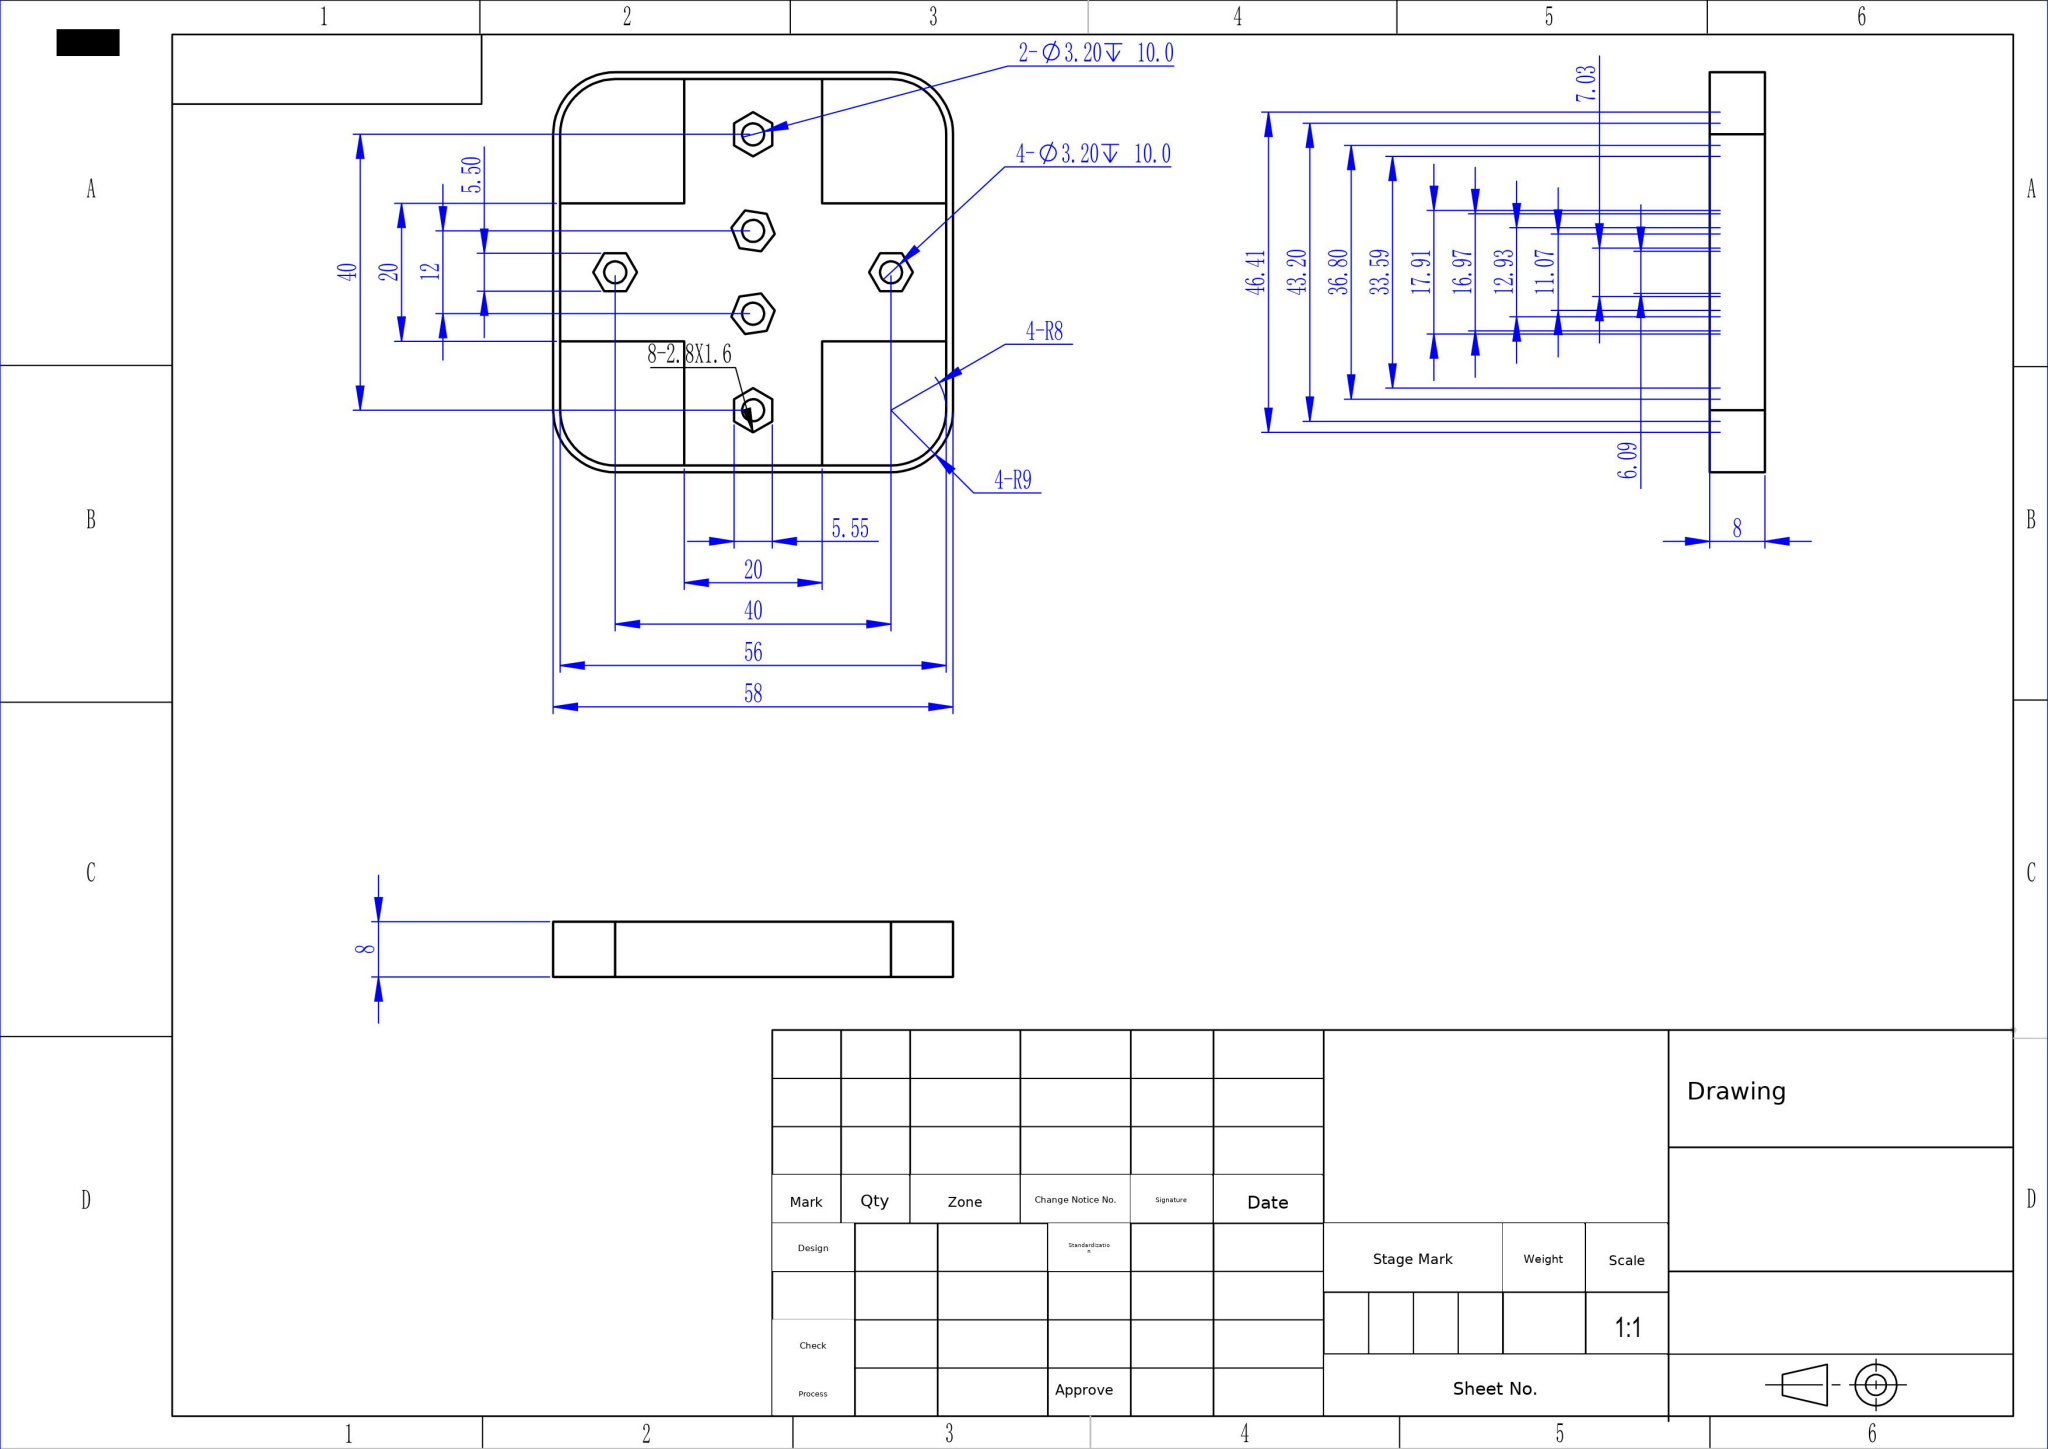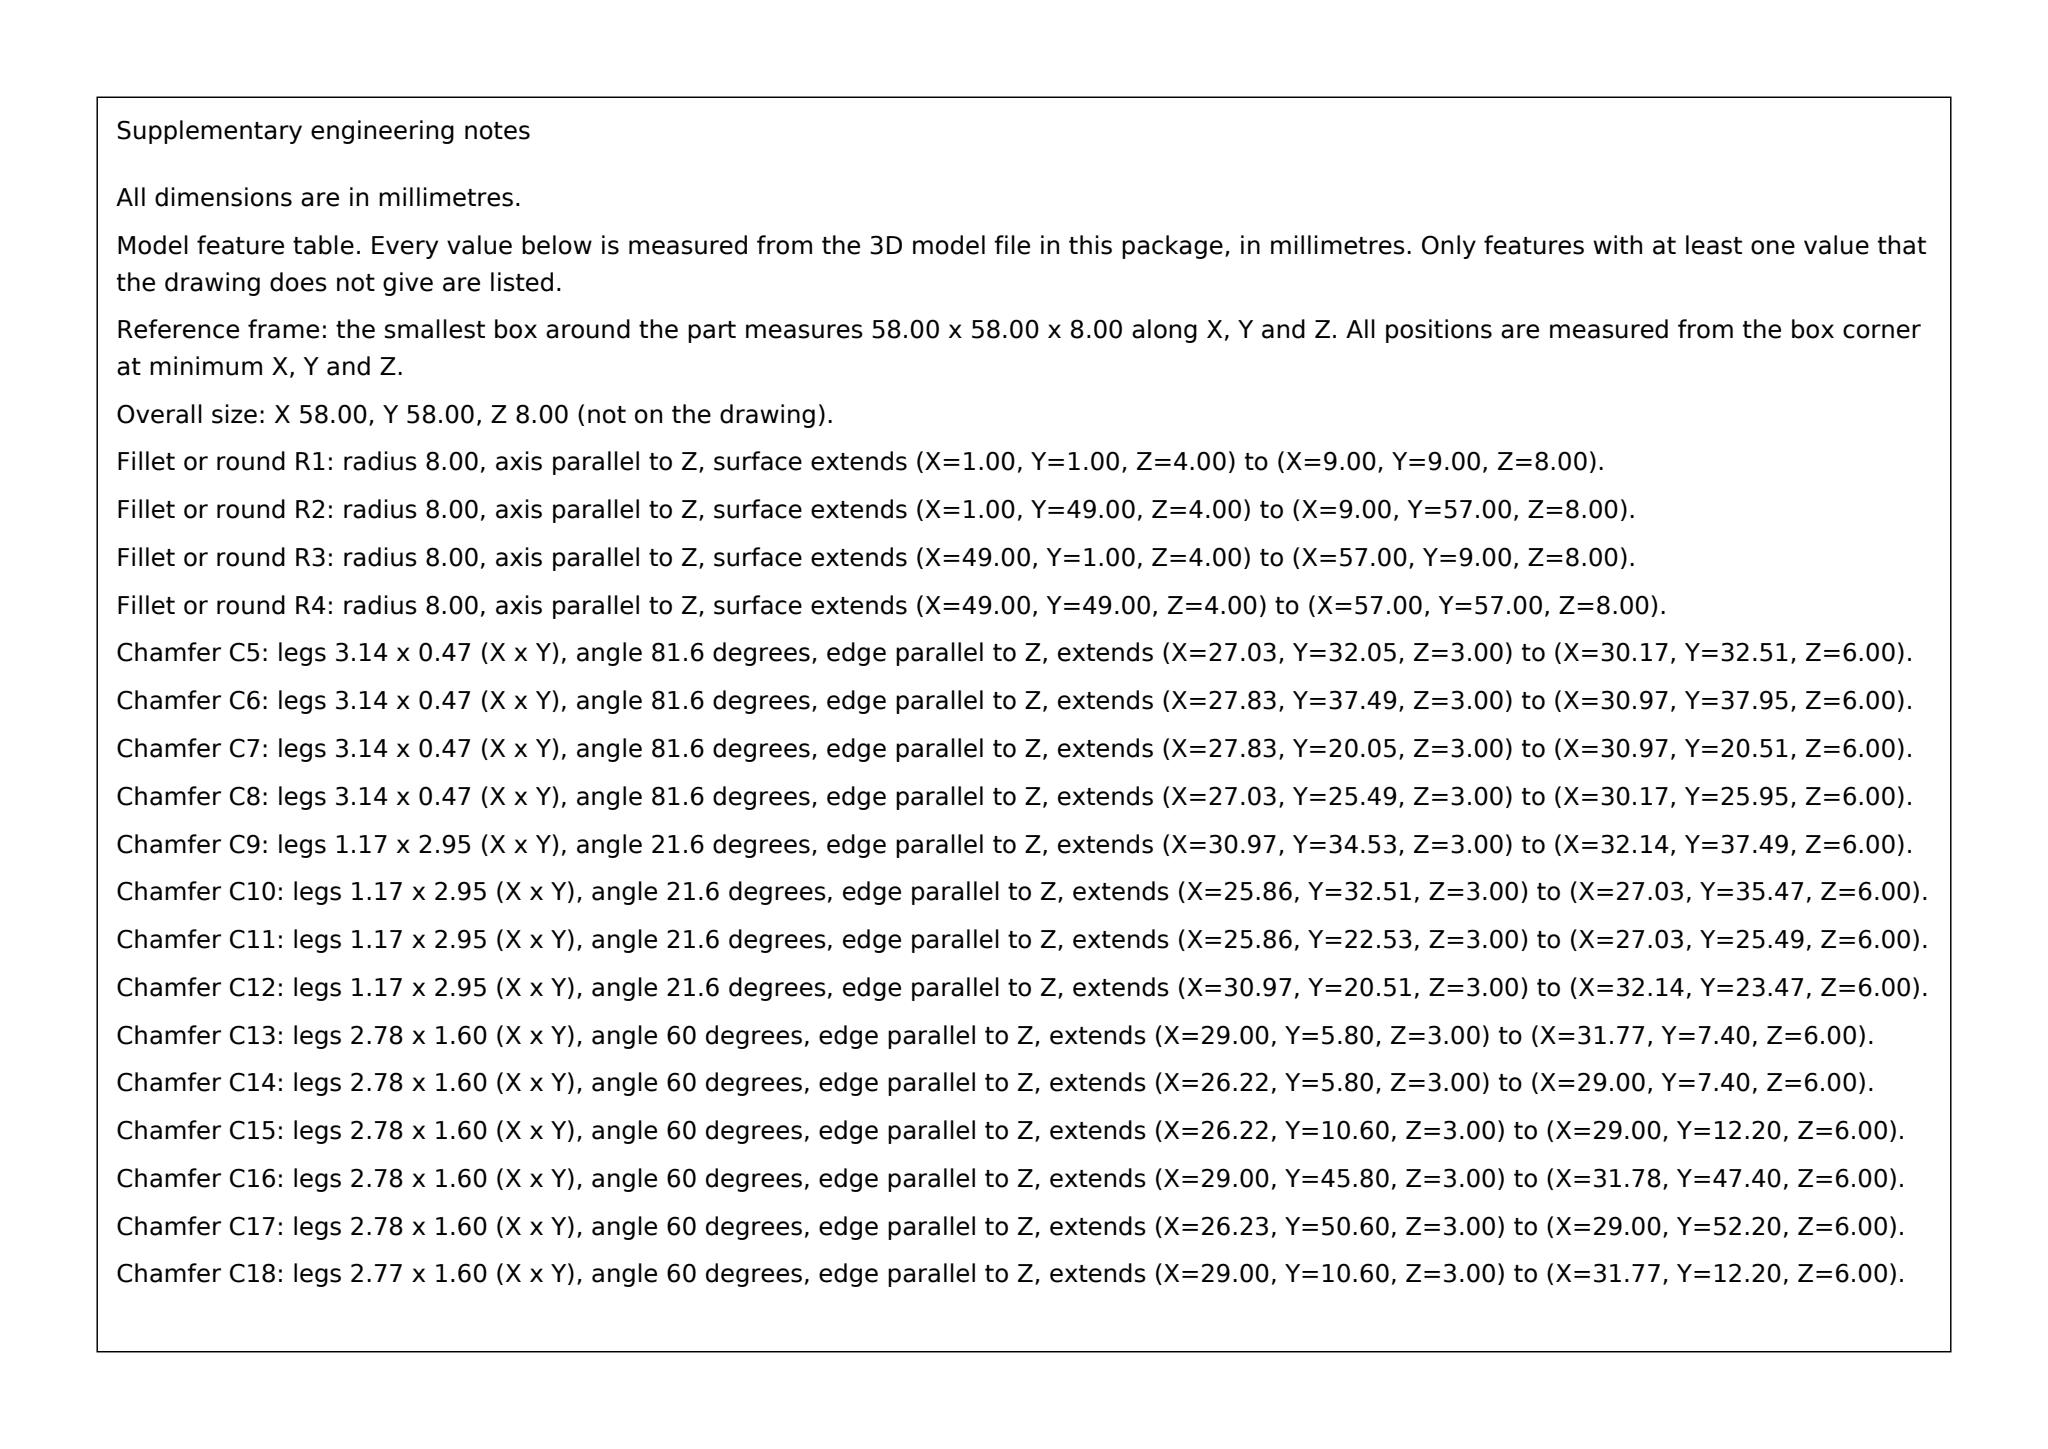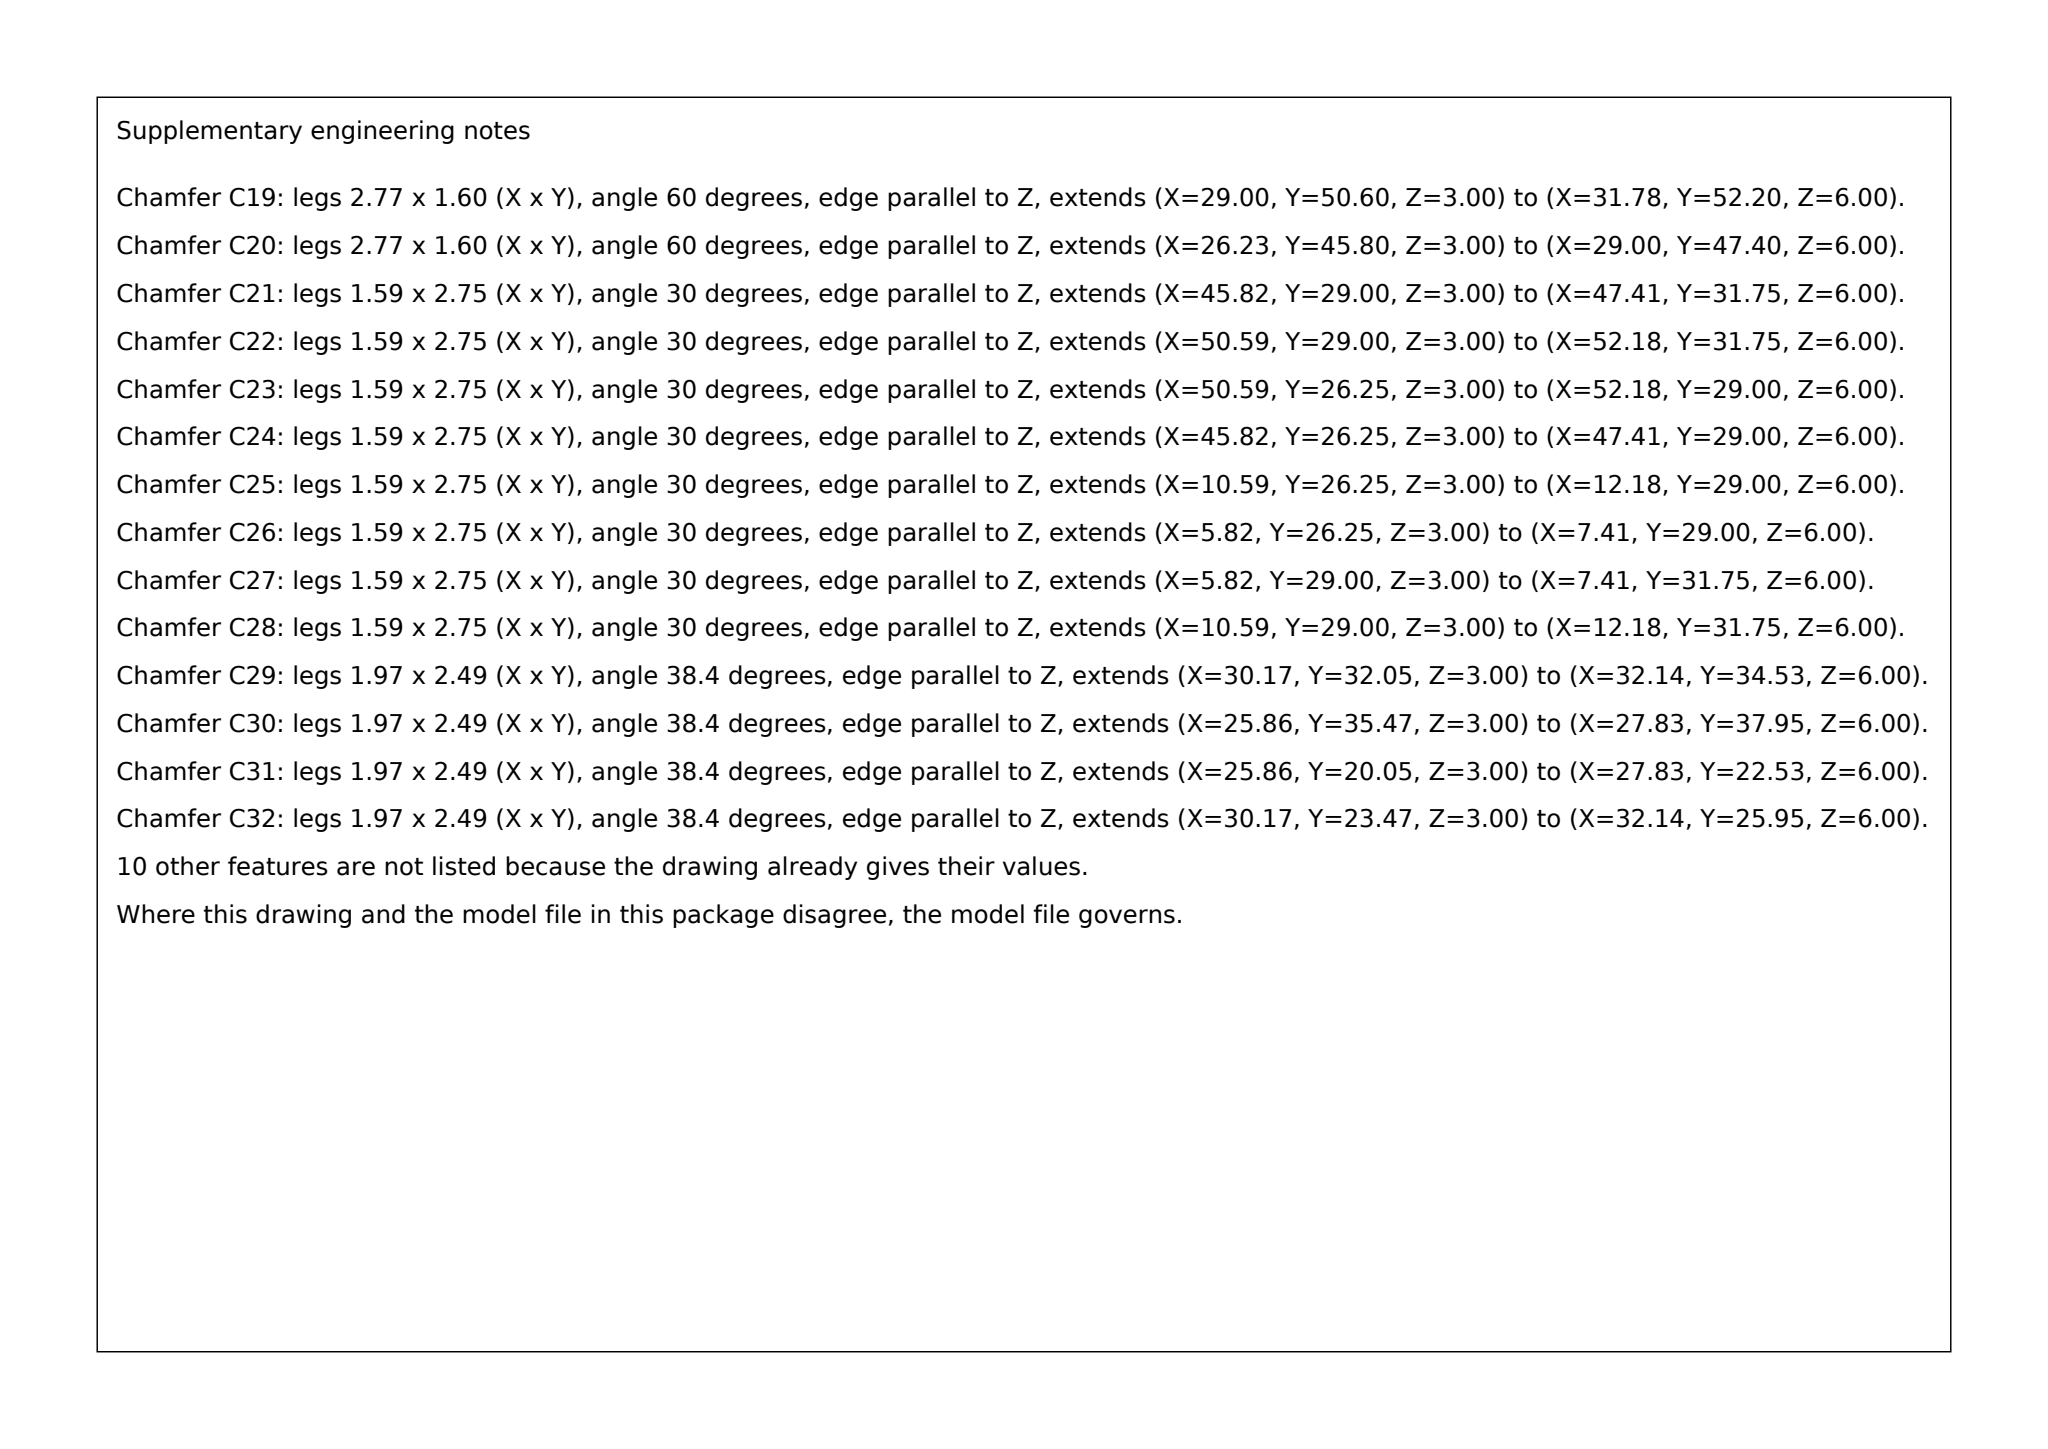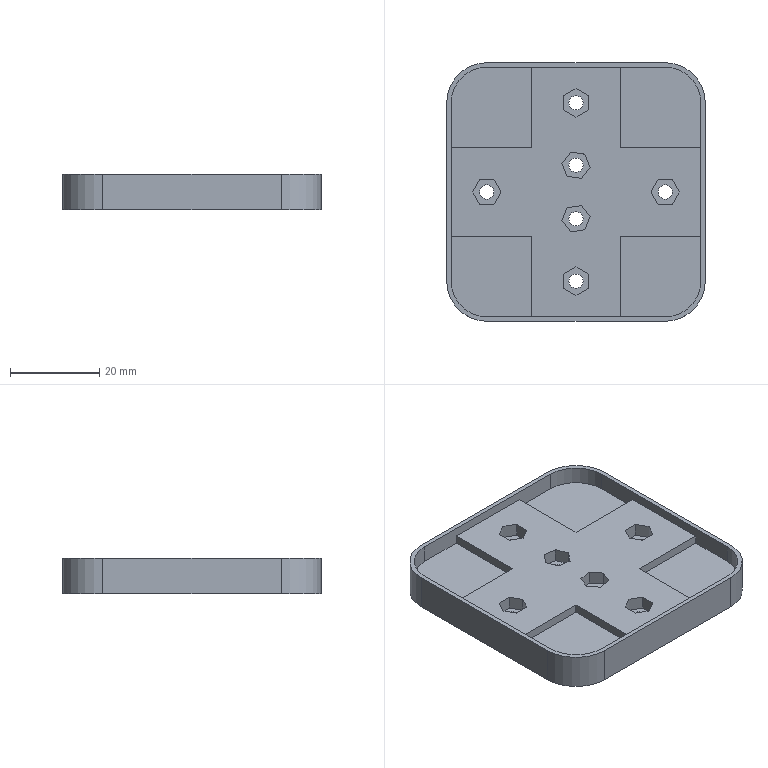Part | SolidWorks | mm | 1 solid | 85 faces | box 58 x 58 x 8 mm | volume 17092 mm3 | plane 65 | cylinder 20 | commonest cylinder face diameters 3.2 x12 18 x4 16 x4
build123d program:
from build123d import *

# Parameters (mm, degrees)
BOSS_EXTRUDE1_DEPTH = 4
BOSS_EXTRUDE2_START = 2
BOSS_EXTRUDE2_DEPTH = 2
BOSS_EXTRUDE3_START = 2
BOSS_EXTRUDE3_DEPTH = 2
SKETCH4_R           = 1.6
CUT_EXTRUDE1_DEPTH  = 10
CUT_EXTRUDE2_DEPTH  = 3
SKETCH7_R           = 1.6
CUT_EXTRUDE3_DEPTH  = 10
CUT_EXTRUDE4_DEPTH  = 3


with BuildPart() as part:
    # Sketch1 → Boss-Extrude1 (new body)
    with BuildSketch(Plane.XY):
        with BuildLine():
            Line((-35.406, 64.537), (4.594, 64.537))
            ThreePointArc((4.594, 64.537), (10.958, 61.901), (13.594, 55.537))
            Line((13.594, 55.537), (13.594, 15.537))
            ThreePointArc((13.594, 15.537), (10.958, 9.173), (4.594, 6.537))
            Line((4.594, 6.537), (-35.406, 6.537))
            ThreePointArc((-35.406, 6.537), (-41.77, 9.173), (-44.406, 15.537))
            Line((-44.406, 15.537), (-44.406, 55.537))
            ThreePointArc((-44.406, 55.537), (-41.77, 61.901), (-35.406, 64.537))
        make_face()
    extrude(amount=-BOSS_EXTRUDE1_DEPTH)

    # Sketch2 → Boss-Extrude2 (add)
    with BuildSketch(Plane.XY.offset(BOSS_EXTRUDE2_START)):
        with BuildLine():
            Line((13.594, 15.537), (13.594, 55.537))
            ThreePointArc((13.594, 55.537), (10.958, 61.901), (4.594, 64.537))
            Line((4.594, 64.537), (-35.406, 64.537))
            ThreePointArc((-35.406, 64.537), (-41.77, 61.901), (-44.406, 55.537))
            Line((-44.406, 55.537), (-44.406, 15.537))
            ThreePointArc((-44.406, 15.537), (-41.77, 9.173), (-35.406, 6.537))
            Line((-35.406, 6.537), (4.594, 6.537))
            ThreePointArc((4.594, 6.537), (10.958, 9.173), (13.594, 15.537))
        make_face()
        with BuildLine():
            Line((-35.406, 63.537), (-25.406, 63.537))
            Line((-25.406, 63.537), (-25.406, 45.537))
            Line((-25.406, 45.537), (-43.406, 45.537))
            Line((-43.406, 45.537), (-43.406, 55.537))
            ThreePointArc((-43.406, 55.537), (-41.063, 61.194), (-35.406, 63.537))
        make_face(mode=Mode.SUBTRACT)
        with BuildLine():
            Line((12.594, 55.537), (12.594, 45.537))
            Line((12.594, 45.537), (-5.406, 45.537))
            Line((-5.406, 45.537), (-5.406, 63.537))
            Line((-5.406, 63.537), (4.594, 63.537))
            ThreePointArc((4.594, 63.537), (10.251, 61.194), (12.594, 55.537))
        make_face(mode=Mode.SUBTRACT)
        with BuildLine():
            Line((-35.406, 7.537), (-25.406, 7.537))
            Line((-25.406, 7.537), (-25.406, 25.537))
            Line((-25.406, 25.537), (-43.406, 25.537))
            Line((-43.406, 25.537), (-43.406, 15.537))
            ThreePointArc((-43.406, 15.537), (-41.063, 9.88), (-35.406, 7.537))
        make_face(mode=Mode.SUBTRACT)
        with BuildLine():
            Line((-5.406, 25.537), (12.594, 25.537))
            Line((12.594, 25.537), (12.594, 15.537))
            ThreePointArc((12.594, 15.537), (10.251, 9.88), (4.594, 7.537))
            Line((4.594, 7.537), (-5.406, 7.537))
            Line((-5.406, 7.537), (-5.406, 25.537))
        make_face(mode=Mode.SUBTRACT)
    extrude(amount=-BOSS_EXTRUDE2_DEPTH)

    # Sketch3 → Boss-Extrude3 (add)
    with BuildSketch(Plane.XY.offset(2).offset(BOSS_EXTRUDE3_START)):
        with BuildLine():
            Line((13.594, 15.537), (13.594, 55.537))
            ThreePointArc((13.594, 55.537), (10.958, 61.901), (4.594, 64.537))
            Line((4.594, 64.537), (-35.406, 64.537))
            ThreePointArc((-35.406, 64.537), (-41.77, 61.901), (-44.406, 55.537))
            Line((-44.406, 55.537), (-44.406, 15.537))
            ThreePointArc((-44.406, 15.537), (-41.77, 9.173), (-35.406, 6.537))
            Line((-35.406, 6.537), (4.594, 6.537))
            ThreePointArc((4.594, 6.537), (10.958, 9.173), (13.594, 15.537))
        make_face()
        with BuildLine():
            Line((-43.406, 55.537), (-43.406, 45.537))
            Line((-43.406, 45.537), (-43.406, 25.537))
            Line((-43.406, 25.537), (-43.406, 15.537))
            ThreePointArc((-43.406, 15.537), (-41.063, 9.88), (-35.406, 7.537))
            Line((-35.406, 7.537), (-25.406, 7.537))
            Line((-25.406, 7.537), (-5.406, 7.537))
            Line((-5.406, 7.537), (4.594, 7.537))
            ThreePointArc((4.594, 7.537), (10.251, 9.88), (12.594, 15.537))
            Line((12.594, 15.537), (12.594, 25.537))
            Line((12.594, 25.537), (12.594, 45.537))
            Line((12.594, 45.537), (12.594, 55.537))
            ThreePointArc((12.594, 55.537), (10.251, 61.194), (4.594, 63.537))
            Line((4.594, 63.537), (-5.406, 63.537))
            Line((-5.406, 63.537), (-25.406, 63.537))
            Line((-25.406, 63.537), (-35.406, 63.537))
            ThreePointArc((-35.406, 63.537), (-41.063, 61.194), (-43.406, 55.537))
        make_face(mode=Mode.SUBTRACT)
    extrude(amount=-BOSS_EXTRUDE3_DEPTH)

    # Sketch4 → Cut-Extrude1 (cut)
    with BuildSketch(Plane.XY.offset(2)):
        with Locations((-15.406, 41.537)):
            Circle(SKETCH4_R)
        with Locations((-15.406, 29.537)):
            Circle(SKETCH4_R)
        with Locations((4.594, 35.537)):
            Circle(SKETCH4_R)
        with Locations((-35.406, 35.537)):
            Circle(SKETCH4_R)
    extrude(amount=-CUT_EXTRUDE1_DEPTH, mode=Mode.SUBTRACT)

    # Sketch5 → Cut-Extrude2 (cut)
    with BuildSketch(Plane.XY.offset(2)):
        Polygon((-13.432, 44.024), (-16.573, 44.49), (-18.547, 42.003), (-17.381, 39.05), (-14.24, 38.584), (-12.265, 41.071), align=None)
        Polygon((1.418, 35.537), (3.006, 32.787), (6.181, 32.787), (7.769, 35.537), (6.181, 38.287), (3.006, 38.287), align=None)
        Polygon((-13.432, 27.05), (-12.265, 30.003), (-14.24, 32.49), (-17.381, 32.024), (-18.547, 29.071), (-16.573, 26.584), align=None)
        Polygon((-32.231, 35.537), (-33.819, 38.287), (-36.994, 38.287), (-38.582, 35.537), (-36.994, 32.787), (-33.819, 32.787), align=None)
    extrude(amount=-CUT_EXTRUDE2_DEPTH, mode=Mode.SUBTRACT)

    # Sketch7 → Cut-Extrude3 (cut)
    with BuildSketch(Plane.XY.offset(2)):
        with Locations((-15.406, 15.537)):
            Circle(SKETCH7_R)
        with Locations((-15.406, 55.537)):
            Circle(SKETCH7_R)
    extrude(amount=-CUT_EXTRUDE3_DEPTH, mode=Mode.SUBTRACT)

    # Sketch8 → Cut-Extrude4 (cut)
    with BuildSketch(Plane.XY.offset(2)):
        Polygon((-15.406, 18.741), (-18.181, 17.139), (-18.181, 13.935), (-15.406, 12.333), (-12.631, 13.935), (-12.631, 17.139), align=None)
        Polygon((-15.406, 58.741), (-18.181, 57.139), (-18.181, 53.935), (-15.406, 52.333), (-12.631, 53.935), (-12.631, 57.139), align=None)
    extrude(amount=-CUT_EXTRUDE4_DEPTH, mode=Mode.SUBTRACT)


solid = part.part